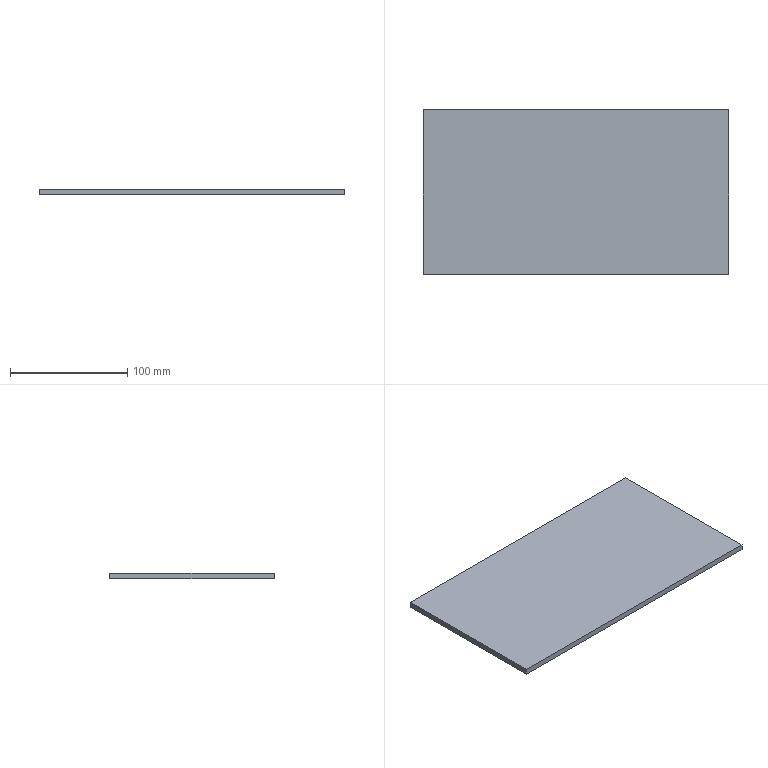Component | SolidWorks | 001UpperConnectingPlate-1 | 1 solid | 6 faces | box 260 x 140 x 5 mm | volume 182000 mm3 | plane 6 | material Plain Carbon Steel
build123d program:
from build123d import *

# Parameters (mm, degrees)
SKETCH1_W           = 260
SKETCH1_H           = 140
BOSS_EXTRUDE1_DEPTH = 5


with BuildPart() as part:
    # Sketch1 → Boss-Extrude1 (new body)
    with BuildSketch(Plane.XY):
        Rectangle(SKETCH1_W, SKETCH1_H)
    extrude(amount=BOSS_EXTRUDE1_DEPTH)


solid = part.part

# Placed as in the assembly
solid = solid.moved(Location((130, 1317, -520), (0, 0, 0)))
STEP:
#1=COLOUR_RGB('',0.7922,0.8196,0.9333);
#2=FILL_AREA_STYLE_COLOUR('',#1);
#3=FILL_AREA_STYLE('',(#2));
#4=SURFACE_STYLE_FILL_AREA(#3);
#5=SURFACE_SIDE_STYLE('',(#4));
#6=SURFACE_STYLE_USAGE(.BOTH.,#5);
#7=PRESENTATION_STYLE_ASSIGNMENT((#6));
#8=CARTESIAN_POINT('',(10.236,49.094,-20.472));
#9=VERTEX_POINT('',#8);
#10=CARTESIAN_POINT('',(10.236,54.606,-20.472));
#11=VERTEX_POINT('',#10);
#12=CARTESIAN_POINT('',(10.236,49.094,-20.472));
#13=DIRECTION('',(0.,1.,0.));
#14=VECTOR('',#13,39.37);
#15=LINE('',#12,#14);
#16=EDGE_CURVE('',#9,#11,#15,.T.);
#17=ORIENTED_EDGE('',*,*,#16,.T.);
#18=CARTESIAN_POINT('',(10.236,54.606,-20.276));
#19=VERTEX_POINT('',#18);
#20=CARTESIAN_POINT('',(10.236,54.606,-20.276));
#21=DIRECTION('',(0.,0.,-1.));
#22=VECTOR('',#21,39.37);
#23=LINE('',#20,#22);
#24=EDGE_CURVE('',#19,#11,#23,.T.);
#25=ORIENTED_EDGE('',*,*,#24,.F.);
#26=CARTESIAN_POINT('',(10.236,49.094,-20.276));
#27=VERTEX_POINT('',#26);
#28=CARTESIAN_POINT('',(10.236,49.094,-20.276));
#29=DIRECTION('',(0.,1.,0.));
#30=VECTOR('',#29,39.37);
#31=LINE('',#28,#30);
#32=EDGE_CURVE('',#27,#19,#31,.T.);
#33=ORIENTED_EDGE('',*,*,#32,.F.);
#34=CARTESIAN_POINT('',(10.236,49.094,-20.276));
#35=DIRECTION('',(0.,0.,-1.));
#36=VECTOR('',#35,39.37);
#37=LINE('',#34,#36);
#38=EDGE_CURVE('',#27,#9,#37,.T.);
#39=ORIENTED_EDGE('',*,*,#38,.T.);
#40=EDGE_LOOP('',(#17,#25,#33,#39));
#41=FACE_OUTER_BOUND('',#40,.T.);
#42=CARTESIAN_POINT('',(10.236,49.094,-20.276));
#43=DIRECTION('',(-1.,0.,0.));
#44=DIRECTION('',(0.,0.,1.));
#45=AXIS2_PLACEMENT_3D('',#42,#43,#44);
#46=PLANE('',#45);
#47=ADVANCED_FACE('',(#41),#46,.F.);
#48=CARTESIAN_POINT('',(0.,54.606,-20.472));
#49=VERTEX_POINT('',#48);
#50=CARTESIAN_POINT('',(0.,54.606,-20.472));
#51=DIRECTION('',(-1.,0.,0.));
#52=VECTOR('',#51,39.37);
#53=LINE('',#50,#52);
#54=EDGE_CURVE('',#11,#49,#53,.T.);
#55=ORIENTED_EDGE('',*,*,#54,.T.);
#56=CARTESIAN_POINT('',(0.,54.606,-20.276));
#57=VERTEX_POINT('',#56);
#58=CARTESIAN_POINT('',(0.,54.606,-20.276));
#59=DIRECTION('',(0.,0.,-1.));
#60=VECTOR('',#59,39.37);
#61=LINE('',#58,#60);
#62=EDGE_CURVE('',#57,#49,#61,.T.);
#63=ORIENTED_EDGE('',*,*,#62,.F.);
#64=CARTESIAN_POINT('',(0.,54.606,-20.276));
#65=DIRECTION('',(-1.,0.,0.));
#66=VECTOR('',#65,39.37);
#67=LINE('',#64,#66);
#68=EDGE_CURVE('',#19,#57,#67,.T.);
#69=ORIENTED_EDGE('',*,*,#68,.F.);
#70=ORIENTED_EDGE('',*,*,#24,.T.);
#71=EDGE_LOOP('',(#55,#63,#69,#70));
#72=FACE_OUTER_BOUND('',#71,.T.);
#73=CARTESIAN_POINT('',(0.,54.606,-20.276));
#74=DIRECTION('',(0.,-1.,0.));
#75=DIRECTION('',(0.,0.,-1.));
#76=AXIS2_PLACEMENT_3D('',#73,#74,#75);
#77=PLANE('',#76);
#78=ADVANCED_FACE('',(#72),#77,.F.);
#79=CARTESIAN_POINT('',(0.,49.094,-20.472));
#80=VERTEX_POINT('',#79);
#81=CARTESIAN_POINT('',(0.,49.094,-20.472));
#82=DIRECTION('',(0.,-1.,0.));
#83=VECTOR('',#82,39.37);
#84=LINE('',#81,#83);
#85=EDGE_CURVE('',#49,#80,#84,.T.);
#86=ORIENTED_EDGE('',*,*,#85,.T.);
#87=CARTESIAN_POINT('',(0.,49.094,-20.276));
#88=VERTEX_POINT('',#87);
#89=CARTESIAN_POINT('',(0.,49.094,-20.276));
#90=DIRECTION('',(0.,0.,-1.));
#91=VECTOR('',#90,39.37);
#92=LINE('',#89,#91);
#93=EDGE_CURVE('',#88,#80,#92,.T.);
#94=ORIENTED_EDGE('',*,*,#93,.F.);
#95=CARTESIAN_POINT('',(0.,49.094,-20.276));
#96=DIRECTION('',(0.,-1.,0.));
#97=VECTOR('',#96,39.37);
#98=LINE('',#95,#97);
#99=EDGE_CURVE('',#57,#88,#98,.T.);
#100=ORIENTED_EDGE('',*,*,#99,.F.);
#101=ORIENTED_EDGE('',*,*,#62,.T.);
#102=EDGE_LOOP('',(#86,#94,#100,#101));
#103=FACE_OUTER_BOUND('',#102,.T.);
#104=CARTESIAN_POINT('',(0.,49.094,-20.276));
#105=DIRECTION('',(1.,0.,0.));
#106=DIRECTION('',(0.,0.,-1.));
#107=AXIS2_PLACEMENT_3D('',#104,#105,#106);
#108=PLANE('',#107);
#109=ADVANCED_FACE('',(#103),#108,.F.);
#110=CARTESIAN_POINT('',(0.,49.094,-20.472));
#111=DIRECTION('',(1.,0.,0.));
#112=VECTOR('',#111,39.37);
#113=LINE('',#110,#112);
#114=EDGE_CURVE('',#80,#9,#113,.T.);
#115=ORIENTED_EDGE('',*,*,#114,.T.);
#116=ORIENTED_EDGE('',*,*,#38,.F.);
#117=CARTESIAN_POINT('',(0.,49.094,-20.276));
#118=DIRECTION('',(1.,0.,0.));
#119=VECTOR('',#118,39.37);
#120=LINE('',#117,#119);
#121=EDGE_CURVE('',#88,#27,#120,.T.);
#122=ORIENTED_EDGE('',*,*,#121,.F.);
#123=ORIENTED_EDGE('',*,*,#93,.T.);
#124=EDGE_LOOP('',(#115,#116,#122,#123));
#125=FACE_OUTER_BOUND('',#124,.T.);
#126=CARTESIAN_POINT('',(0.,49.094,-20.276));
#127=DIRECTION('',(0.,1.,0.));
#128=DIRECTION('',(0.,0.,1.));
#129=AXIS2_PLACEMENT_3D('',#126,#127,#128);
#130=PLANE('',#129);
#131=ADVANCED_FACE('',(#125),#130,.F.);
#132=ORIENTED_EDGE('',*,*,#32,.T.);
#133=ORIENTED_EDGE('',*,*,#68,.T.);
#134=ORIENTED_EDGE('',*,*,#99,.T.);
#135=ORIENTED_EDGE('',*,*,#121,.T.);
#136=EDGE_LOOP('',(#132,#133,#134,#135));
#137=FACE_OUTER_BOUND('',#136,.T.);
#138=CARTESIAN_POINT('',(10.236,54.606,-20.276));
#139=DIRECTION('',(0.,0.,-1.));
#140=DIRECTION('',(-1.,0.,0.));
#141=AXIS2_PLACEMENT_3D('',#138,#139,#140);
#142=PLANE('',#141);
#143=ADVANCED_FACE('',(#137),#142,.F.);
#144=ORIENTED_EDGE('',*,*,#16,.F.);
#145=ORIENTED_EDGE('',*,*,#114,.F.);
#146=ORIENTED_EDGE('',*,*,#85,.F.);
#147=ORIENTED_EDGE('',*,*,#54,.F.);
#148=EDGE_LOOP('',(#144,#145,#146,#147));
#149=FACE_OUTER_BOUND('',#148,.T.);
#150=CARTESIAN_POINT('',(10.236,54.606,-20.472));
#151=DIRECTION('',(0.,0.,-1.));
#152=DIRECTION('',(-1.,0.,0.));
#153=AXIS2_PLACEMENT_3D('',#150,#151,#152);
#154=PLANE('',#153);
#155=ADVANCED_FACE('',(#149),#154,.T.);
#156=CLOSED_SHELL('',(#47,#78,#109,#131,#143,#155));
#157=MANIFOLD_SOLID_BREP('',#156);
#158=STYLED_ITEM('',(#7),#157);
#159=PRESENTATION_LAYER_ASSIGNMENT('','',(#158));
#160=CARTESIAN_POINT('',(0.,0.,0.));
#161=DIRECTION('',(0.,0.,1.));
#162=DIRECTION('',(1.,0.,0.));
#163=AXIS2_PLACEMENT_3D('',#160,#161,#162);
#164=(LENGTH_UNIT()NAMED_UNIT(*)SI_UNIT($,.METRE.));
#165=LENGTH_MEASURE_WITH_UNIT(LENGTH_MEASURE(0.0254),#164);
#166=DIMENSIONAL_EXPONENTS(1.,0.,0.,0.,0.,0.,0.);
#167=(CONVERSION_BASED_UNIT('',#165)LENGTH_UNIT()NAMED_UNIT(#166));
#168=UNCERTAINTY_MEASURE_WITH_UNIT(LENGTH_MEASURE(0.00001),#167,'','');
#169=(NAMED_UNIT(*)PLANE_ANGLE_UNIT()SI_UNIT($,.RADIAN.));
#170=(NAMED_UNIT(*)SI_UNIT($,.STERADIAN.)SOLID_ANGLE_UNIT());
#171=(GEOMETRIC_REPRESENTATION_CONTEXT(3)GLOBAL_UNCERTAINTY_ASSIGNED_CONTEXT((#168))GLOBAL_UNIT_ASSIGNED_CONTEXT((#167,#169,#170))REPRESENTATION_CONTEXT('',''));
#172=ADVANCED_BREP_SHAPE_REPRESENTATION('',(#157,#163),#171);
#173=(LENGTH_UNIT()NAMED_UNIT(*)SI_UNIT($,.METRE.));
#174=LENGTH_MEASURE_WITH_UNIT(LENGTH_MEASURE(0.0254),#173);
#175=DIMENSIONAL_EXPONENTS(1.,0.,0.,0.,0.,0.,0.);
#176=(CONVERSION_BASED_UNIT('',#174)LENGTH_UNIT()NAMED_UNIT(#175));
#177=UNCERTAINTY_MEASURE_WITH_UNIT(LENGTH_MEASURE(0.00001),#176,'','');
#178=(NAMED_UNIT(*)PLANE_ANGLE_UNIT()SI_UNIT($,.RADIAN.));
#179=(NAMED_UNIT(*)SI_UNIT($,.STERADIAN.)SOLID_ANGLE_UNIT());
#180=(GEOMETRIC_REPRESENTATION_CONTEXT(3)GLOBAL_UNCERTAINTY_ASSIGNED_CONTEXT((#177))GLOBAL_UNIT_ASSIGNED_CONTEXT((#176,#178,#179))REPRESENTATION_CONTEXT('',''));
#181=MECHANICAL_DESIGN_GEOMETRIC_PRESENTATION_REPRESENTATION('',(#158),#180);